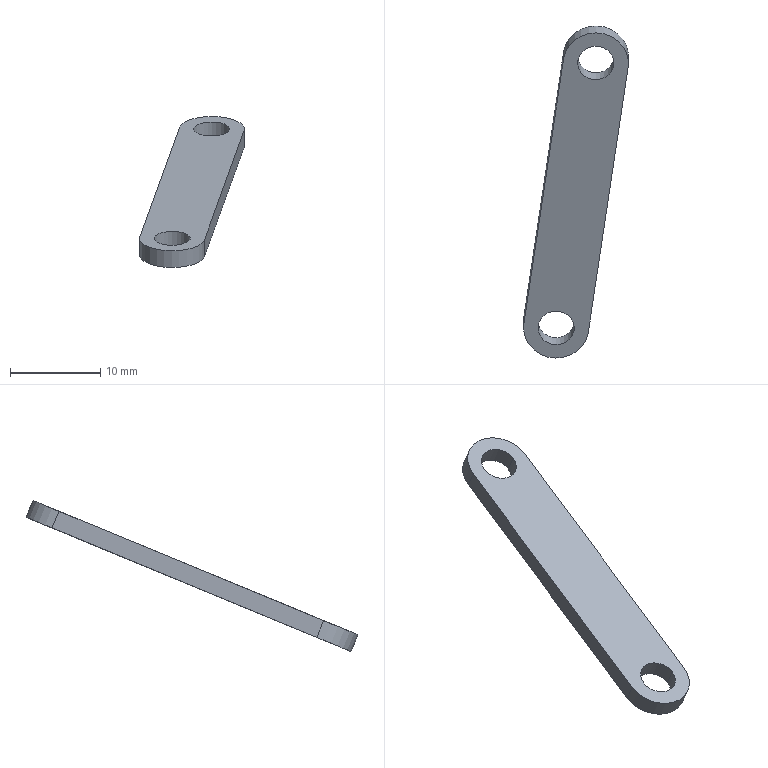Component | SolidWorks | Long Arm-1 | 1 solid | 10 faces | box 11.59 x 36.71 x 16.7 mm | volume 492 mm3 | cylinder 6 | plane 4 | commonest cylinder face diameters 4 x4 7.2 x2
build123d program:
from build123d import *

# Parameters (mm, degrees)
SKETCH2_R           = 5
BOSS_EXTRUDE1_DEPTH = 2.5
SCALE1_SCALE        = 0.4


with BuildPart() as part:
    # Sketch2 → Boss-Extrude1 (new, symmetric)
    with BuildSketch(Plane(origin=(0, 0, 0), x_dir=(1, 0, 0), z_dir=(0, 1, 0))):
        with BuildLine():
            Line((0, 9), (80, 9))
            ThreePointArc((80, 9), (89, 0), (80, -9))
            Line((80, -9), (0, -9))
            ThreePointArc((0, -9), (-9, 0), (0, 9))
        make_face()
        with Locations(Location((0, 0, 0), (0, 0, 270))):
            Circle(SKETCH2_R, mode=Mode.SUBTRACT)
        with Locations(Location((80, 0, 0), (0, 0, 270))):
            Circle(SKETCH2_R, mode=Mode.SUBTRACT)
    extrude(amount=BOSS_EXTRUDE1_DEPTH, both=True)


with BuildPart() as part_1:
    # Scale1: scaled about (0, 0, 0)
    add(part.part.scale(SCALE1_SCALE))


solid = part_1.part

# Placed as in the assembly
solid = solid.moved(Location((343.013, 24.265, 76.802), (-67.552, -82.111, 180)))
STEP:
#1=CARTESIAN_POINT('',(13.582,0.9604,2.983));
#2=VERTEX_POINT('',#1);
#3=CARTESIAN_POINT('',(13.426,0.9803,2.991));
#4=VERTEX_POINT('',#3);
#5=CARTESIAN_POINT('',(13.504,0.9703,2.987));
#6=DIRECTION('',(0.,0.3818,-0.9242));
#7=DIRECTION('',(-0.9905,0.1268,0.05241));
#8=AXIS2_PLACEMENT_3D('',#5,#6,#7);
#9=CIRCLE('',#8,0.07874);
#10=EDGE_CURVE('',#2,#4,#9,.T.);
#11=ORIENTED_EDGE('',*,*,#10,.T.);
#12=CARTESIAN_POINT('',(13.426,0.9503,3.064));
#13=VERTEX_POINT('',#12);
#14=CARTESIAN_POINT('',(13.426,0.9803,2.991));
#15=DIRECTION('',(-0.,-0.3818,0.9242));
#16=VECTOR('',#15,39.37);
#17=LINE('',#14,#16);
#18=EDGE_CURVE('',#4,#13,#17,.T.);
#19=ORIENTED_EDGE('',*,*,#18,.T.);
#20=CARTESIAN_POINT('',(13.582,0.9303,3.056));
#21=VERTEX_POINT('',#20);
#22=CARTESIAN_POINT('',(13.504,0.9403,3.06));
#23=DIRECTION('',(0.,0.3818,-0.9242));
#24=DIRECTION('',(-0.9905,0.1268,0.05241));
#25=AXIS2_PLACEMENT_3D('',#22,#23,#24);
#26=CIRCLE('',#25,0.07874);
#27=EDGE_CURVE('',#21,#13,#26,.T.);
#28=ORIENTED_EDGE('',*,*,#27,.F.);
#29=CARTESIAN_POINT('',(13.582,0.9604,2.983));
#30=DIRECTION('',(-0.,-0.3818,0.9242));
#31=VECTOR('',#30,39.37);
#32=LINE('',#29,#31);
#33=EDGE_CURVE('',#2,#21,#32,.T.);
#34=ORIENTED_EDGE('',*,*,#33,.F.);
#35=EDGE_LOOP('',(#11,#19,#28,#34));
#36=FACE_OUTER_BOUND('',#35,.T.);
#37=CARTESIAN_POINT('',(13.504,0.9703,2.987));
#38=DIRECTION('',(-0.,-0.3818,0.9242));
#39=DIRECTION('',(0.9905,-0.1268,-0.05241));
#40=AXIS2_PLACEMENT_3D('',#37,#38,#39);
#41=CYLINDRICAL_SURFACE('',#40,0.07874);
#42=ADVANCED_FACE('',(#36),#41,.F.);
#43=CARTESIAN_POINT('',(13.41,-0.193,2.507));
#44=VERTEX_POINT('',#43);
#45=CARTESIAN_POINT('',(13.254,-0.173,2.515));
#46=VERTEX_POINT('',#45);
#47=CARTESIAN_POINT('',(13.332,-0.183,2.511));
#48=DIRECTION('',(0.,0.3818,-0.9242));
#49=DIRECTION('',(-0.9905,0.1268,0.05241));
#50=AXIS2_PLACEMENT_3D('',#47,#48,#49);
#51=CIRCLE('',#50,0.07874);
#52=EDGE_CURVE('',#44,#46,#51,.T.);
#53=ORIENTED_EDGE('',*,*,#52,.T.);
#54=CARTESIAN_POINT('',(13.254,-0.2031,2.588));
#55=VERTEX_POINT('',#54);
#56=CARTESIAN_POINT('',(13.254,-0.173,2.515));
#57=DIRECTION('',(-0.,-0.3818,0.9242));
#58=VECTOR('',#57,39.37);
#59=LINE('',#56,#58);
#60=EDGE_CURVE('',#46,#55,#59,.T.);
#61=ORIENTED_EDGE('',*,*,#60,.T.);
#62=CARTESIAN_POINT('',(13.41,-0.2231,2.579));
#63=VERTEX_POINT('',#62);
#64=CARTESIAN_POINT('',(13.332,-0.2131,2.584));
#65=DIRECTION('',(0.,0.3818,-0.9242));
#66=DIRECTION('',(-0.9905,0.1268,0.05241));
#67=AXIS2_PLACEMENT_3D('',#64,#65,#66);
#68=CIRCLE('',#67,0.07874);
#69=EDGE_CURVE('',#63,#55,#68,.T.);
#70=ORIENTED_EDGE('',*,*,#69,.F.);
#71=CARTESIAN_POINT('',(13.41,-0.193,2.507));
#72=DIRECTION('',(-0.,-0.3818,0.9242));
#73=VECTOR('',#72,39.37);
#74=LINE('',#71,#73);
#75=EDGE_CURVE('',#44,#63,#74,.T.);
#76=ORIENTED_EDGE('',*,*,#75,.F.);
#77=EDGE_LOOP('',(#53,#61,#70,#76));
#78=FACE_OUTER_BOUND('',#77,.T.);
#79=CARTESIAN_POINT('',(13.332,-0.183,2.511));
#80=DIRECTION('',(-0.,-0.3818,0.9242));
#81=DIRECTION('',(0.9905,-0.1268,-0.05241));
#82=AXIS2_PLACEMENT_3D('',#79,#80,#81);
#83=CYLINDRICAL_SURFACE('',#82,0.07874);
#84=ADVANCED_FACE('',(#78),#83,.F.);
#85=ORIENTED_EDGE('',*,*,#52,.F.);
#86=CARTESIAN_POINT('',(13.332,-0.183,2.511));
#87=DIRECTION('',(0.,0.3818,-0.9242));
#88=DIRECTION('',(-0.9905,0.1268,0.05241));
#89=AXIS2_PLACEMENT_3D('',#86,#87,#88);
#90=CIRCLE('',#89,0.07874);
#91=EDGE_CURVE('',#46,#44,#90,.T.);
#92=ORIENTED_EDGE('',*,*,#91,.F.);
#93=EDGE_LOOP('',(#85,#92));
#94=FACE_BOUND('',#93,.T.);
#95=CARTESIAN_POINT('',(13.472,-0.201,2.503));
#96=VERTEX_POINT('',#95);
#97=CARTESIAN_POINT('',(13.191,-0.165,2.518));
#98=VERTEX_POINT('',#97);
#99=CARTESIAN_POINT('',(13.332,-0.183,2.511));
#100=DIRECTION('',(0.,0.3818,-0.9242));
#101=DIRECTION('',(-0.9905,0.1268,0.05241));
#102=AXIS2_PLACEMENT_3D('',#99,#100,#101);
#103=CIRCLE('',#102,0.1417);
#104=EDGE_CURVE('',#96,#98,#103,.T.);
#105=ORIENTED_EDGE('',*,*,#104,.T.);
#106=CARTESIAN_POINT('',(13.364,0.9883,2.995));
#107=VERTEX_POINT('',#106);
#108=CARTESIAN_POINT('',(13.191,-0.165,2.518));
#109=DIRECTION('',(0.1372,0.9155,0.3782));
#110=VECTOR('',#109,39.37);
#111=LINE('',#108,#110);
#112=EDGE_CURVE('',#98,#107,#111,.T.);
#113=ORIENTED_EDGE('',*,*,#112,.T.);
#114=CARTESIAN_POINT('',(13.645,0.9524,2.98));
#115=VERTEX_POINT('',#114);
#116=CARTESIAN_POINT('',(13.504,0.9703,2.987));
#117=DIRECTION('',(0.,0.3818,-0.9242));
#118=DIRECTION('',(-0.9905,0.1268,0.05241));
#119=AXIS2_PLACEMENT_3D('',#116,#117,#118);
#120=CIRCLE('',#119,0.1417);
#121=EDGE_CURVE('',#107,#115,#120,.T.);
#122=ORIENTED_EDGE('',*,*,#121,.T.);
#123=CARTESIAN_POINT('',(13.472,-0.201,2.503));
#124=DIRECTION('',(-0.1372,-0.9155,-0.3782));
#125=VECTOR('',#124,39.37);
#126=LINE('',#123,#125);
#127=EDGE_CURVE('',#115,#96,#126,.T.);
#128=ORIENTED_EDGE('',*,*,#127,.T.);
#129=EDGE_LOOP('',(#105,#113,#122,#128));
#130=FACE_OUTER_BOUND('',#129,.T.);
#131=ORIENTED_EDGE('',*,*,#10,.F.);
#132=CARTESIAN_POINT('',(13.504,0.9703,2.987));
#133=DIRECTION('',(0.,0.3818,-0.9242));
#134=DIRECTION('',(-0.9905,0.1268,0.05241));
#135=AXIS2_PLACEMENT_3D('',#132,#133,#134);
#136=CIRCLE('',#135,0.07874);
#137=EDGE_CURVE('',#4,#2,#136,.T.);
#138=ORIENTED_EDGE('',*,*,#137,.F.);
#139=EDGE_LOOP('',(#131,#138));
#140=FACE_BOUND('',#139,.T.);
#141=CARTESIAN_POINT('',(13.332,-0.183,2.511));
#142=DIRECTION('',(0.,0.3818,-0.9242));
#143=DIRECTION('',(-0.9905,0.1268,0.05241));
#144=AXIS2_PLACEMENT_3D('',#141,#142,#143);
#145=PLANE('',#144);
#146=ADVANCED_FACE('',(#94,#130,#140),#145,.T.);
#147=CARTESIAN_POINT('',(13.472,-0.2311,2.576));
#148=VERTEX_POINT('',#147);
#149=CARTESIAN_POINT('',(13.191,-0.1951,2.591));
#150=VERTEX_POINT('',#149);
#151=CARTESIAN_POINT('',(13.332,-0.2131,2.584));
#152=DIRECTION('',(0.,0.3818,-0.9242));
#153=DIRECTION('',(-0.9905,0.1268,0.05241));
#154=AXIS2_PLACEMENT_3D('',#151,#152,#153);
#155=CIRCLE('',#154,0.1417);
#156=EDGE_CURVE('',#148,#150,#155,.T.);
#157=ORIENTED_EDGE('',*,*,#156,.F.);
#158=CARTESIAN_POINT('',(13.645,0.9223,3.053));
#159=VERTEX_POINT('',#158);
#160=CARTESIAN_POINT('',(13.472,-0.2311,2.576));
#161=DIRECTION('',(-0.1372,-0.9155,-0.3782));
#162=VECTOR('',#161,39.37);
#163=LINE('',#160,#162);
#164=EDGE_CURVE('',#159,#148,#163,.T.);
#165=ORIENTED_EDGE('',*,*,#164,.F.);
#166=CARTESIAN_POINT('',(13.364,0.9583,3.068));
#167=VERTEX_POINT('',#166);
#168=CARTESIAN_POINT('',(13.504,0.9403,3.06));
#169=DIRECTION('',(0.,0.3818,-0.9242));
#170=DIRECTION('',(-0.9905,0.1268,0.05241));
#171=AXIS2_PLACEMENT_3D('',#168,#169,#170);
#172=CIRCLE('',#171,0.1417);
#173=EDGE_CURVE('',#167,#159,#172,.T.);
#174=ORIENTED_EDGE('',*,*,#173,.F.);
#175=CARTESIAN_POINT('',(13.191,-0.1951,2.591));
#176=DIRECTION('',(0.1372,0.9155,0.3782));
#177=VECTOR('',#176,39.37);
#178=LINE('',#175,#177);
#179=EDGE_CURVE('',#150,#167,#178,.T.);
#180=ORIENTED_EDGE('',*,*,#179,.F.);
#181=EDGE_LOOP('',(#157,#165,#174,#180));
#182=FACE_OUTER_BOUND('',#181,.T.);
#183=ORIENTED_EDGE('',*,*,#69,.T.);
#184=CARTESIAN_POINT('',(13.332,-0.2131,2.584));
#185=DIRECTION('',(0.,0.3818,-0.9242));
#186=DIRECTION('',(-0.9905,0.1268,0.05241));
#187=AXIS2_PLACEMENT_3D('',#184,#185,#186);
#188=CIRCLE('',#187,0.07874);
#189=EDGE_CURVE('',#55,#63,#188,.T.);
#190=ORIENTED_EDGE('',*,*,#189,.T.);
#191=EDGE_LOOP('',(#183,#190));
#192=FACE_BOUND('',#191,.T.);
#193=ORIENTED_EDGE('',*,*,#27,.T.);
#194=CARTESIAN_POINT('',(13.504,0.9403,3.06));
#195=DIRECTION('',(0.,0.3818,-0.9242));
#196=DIRECTION('',(-0.9905,0.1268,0.05241));
#197=AXIS2_PLACEMENT_3D('',#194,#195,#196);
#198=CIRCLE('',#197,0.07874);
#199=EDGE_CURVE('',#13,#21,#198,.T.);
#200=ORIENTED_EDGE('',*,*,#199,.T.);
#201=EDGE_LOOP('',(#193,#200));
#202=FACE_BOUND('',#201,.T.);
#203=CARTESIAN_POINT('',(13.332,-0.2131,2.584));
#204=DIRECTION('',(0.,0.3818,-0.9242));
#205=DIRECTION('',(-0.9905,0.1268,0.05241));
#206=AXIS2_PLACEMENT_3D('',#203,#204,#205);
#207=PLANE('',#206);
#208=ADVANCED_FACE('',(#182,#192,#202),#207,.F.);
#209=ORIENTED_EDGE('',*,*,#156,.T.);
#210=CARTESIAN_POINT('',(13.191,-0.165,2.518));
#211=DIRECTION('',(-0.,-0.3818,0.9242));
#212=VECTOR('',#211,39.37);
#213=LINE('',#210,#212);
#214=EDGE_CURVE('',#98,#150,#213,.T.);
#215=ORIENTED_EDGE('',*,*,#214,.F.);
#216=ORIENTED_EDGE('',*,*,#104,.F.);
#217=CARTESIAN_POINT('',(13.472,-0.201,2.503));
#218=DIRECTION('',(-0.,-0.3818,0.9242));
#219=VECTOR('',#218,39.37);
#220=LINE('',#217,#219);
#221=EDGE_CURVE('',#96,#148,#220,.T.);
#222=ORIENTED_EDGE('',*,*,#221,.T.);
#223=EDGE_LOOP('',(#209,#215,#216,#222));
#224=FACE_OUTER_BOUND('',#223,.T.);
#225=CARTESIAN_POINT('',(13.332,-0.183,2.511));
#226=DIRECTION('',(-0.,-0.3818,0.9242));
#227=DIRECTION('',(0.9905,-0.1268,-0.05241));
#228=AXIS2_PLACEMENT_3D('',#225,#226,#227);
#229=CYLINDRICAL_SURFACE('',#228,0.1417);
#230=ADVANCED_FACE('',(#224),#229,.T.);
#231=ORIENTED_EDGE('',*,*,#179,.T.);
#232=CARTESIAN_POINT('',(13.364,0.9883,2.995));
#233=DIRECTION('',(-0.,-0.3818,0.9242));
#234=VECTOR('',#233,39.37);
#235=LINE('',#232,#234);
#236=EDGE_CURVE('',#107,#167,#235,.T.);
#237=ORIENTED_EDGE('',*,*,#236,.F.);
#238=ORIENTED_EDGE('',*,*,#112,.F.);
#239=ORIENTED_EDGE('',*,*,#214,.T.);
#240=EDGE_LOOP('',(#231,#237,#238,#239));
#241=FACE_OUTER_BOUND('',#240,.T.);
#242=CARTESIAN_POINT('',(13.191,-0.165,2.518));
#243=DIRECTION('',(0.9905,-0.1268,-0.05241));
#244=DIRECTION('',(-0.1372,-0.9155,-0.3782));
#245=AXIS2_PLACEMENT_3D('',#242,#243,#244);
#246=PLANE('',#245);
#247=ADVANCED_FACE('',(#241),#246,.F.);
#248=ORIENTED_EDGE('',*,*,#173,.T.);
#249=CARTESIAN_POINT('',(13.645,0.9524,2.98));
#250=DIRECTION('',(-0.,-0.3818,0.9242));
#251=VECTOR('',#250,39.37);
#252=LINE('',#249,#251);
#253=EDGE_CURVE('',#115,#159,#252,.T.);
#254=ORIENTED_EDGE('',*,*,#253,.F.);
#255=ORIENTED_EDGE('',*,*,#121,.F.);
#256=ORIENTED_EDGE('',*,*,#236,.T.);
#257=EDGE_LOOP('',(#248,#254,#255,#256));
#258=FACE_OUTER_BOUND('',#257,.T.);
#259=CARTESIAN_POINT('',(13.504,0.9703,2.987));
#260=DIRECTION('',(-0.,-0.3818,0.9242));
#261=DIRECTION('',(0.9905,-0.1268,-0.05241));
#262=AXIS2_PLACEMENT_3D('',#259,#260,#261);
#263=CYLINDRICAL_SURFACE('',#262,0.1417);
#264=ADVANCED_FACE('',(#258),#263,.T.);
#265=ORIENTED_EDGE('',*,*,#164,.T.);
#266=ORIENTED_EDGE('',*,*,#221,.F.);
#267=ORIENTED_EDGE('',*,*,#127,.F.);
#268=ORIENTED_EDGE('',*,*,#253,.T.);
#269=EDGE_LOOP('',(#265,#266,#267,#268));
#270=FACE_OUTER_BOUND('',#269,.T.);
#271=CARTESIAN_POINT('',(13.472,-0.201,2.503));
#272=DIRECTION('',(-0.9905,0.1268,0.05241));
#273=DIRECTION('',(0.1372,0.9155,0.3782));
#274=AXIS2_PLACEMENT_3D('',#271,#272,#273);
#275=PLANE('',#274);
#276=ADVANCED_FACE('',(#270),#275,.F.);
#277=ORIENTED_EDGE('',*,*,#60,.F.);
#278=ORIENTED_EDGE('',*,*,#91,.T.);
#279=ORIENTED_EDGE('',*,*,#75,.T.);
#280=ORIENTED_EDGE('',*,*,#189,.F.);
#281=EDGE_LOOP('',(#277,#278,#279,#280));
#282=FACE_OUTER_BOUND('',#281,.T.);
#283=CARTESIAN_POINT('',(13.332,-0.183,2.511));
#284=DIRECTION('',(-0.,-0.3818,0.9242));
#285=DIRECTION('',(0.9905,-0.1268,-0.05241));
#286=AXIS2_PLACEMENT_3D('',#283,#284,#285);
#287=CYLINDRICAL_SURFACE('',#286,0.07874);
#288=ADVANCED_FACE('',(#282),#287,.F.);
#289=ORIENTED_EDGE('',*,*,#18,.F.);
#290=ORIENTED_EDGE('',*,*,#137,.T.);
#291=ORIENTED_EDGE('',*,*,#33,.T.);
#292=ORIENTED_EDGE('',*,*,#199,.F.);
#293=EDGE_LOOP('',(#289,#290,#291,#292));
#294=FACE_OUTER_BOUND('',#293,.T.);
#295=CARTESIAN_POINT('',(13.504,0.9703,2.987));
#296=DIRECTION('',(-0.,-0.3818,0.9242));
#297=DIRECTION('',(0.9905,-0.1268,-0.05241));
#298=AXIS2_PLACEMENT_3D('',#295,#296,#297);
#299=CYLINDRICAL_SURFACE('',#298,0.07874);
#300=ADVANCED_FACE('',(#294),#299,.F.);
#301=CLOSED_SHELL('',(#42,#84,#146,#208,#230,#247,#264,#276,#288,#300));
#302=MANIFOLD_SOLID_BREP('',#301);
#303=CARTESIAN_POINT('',(0.,0.,0.));
#304=DIRECTION('',(0.,0.,1.));
#305=DIRECTION('',(1.,0.,0.));
#306=AXIS2_PLACEMENT_3D('',#303,#304,#305);
#307=(LENGTH_UNIT()NAMED_UNIT(*)SI_UNIT($,.METRE.));
#308=LENGTH_MEASURE_WITH_UNIT(LENGTH_MEASURE(0.0254),#307);
#309=DIMENSIONAL_EXPONENTS(1.,0.,0.,0.,0.,0.,0.);
#310=(CONVERSION_BASED_UNIT('',#308)LENGTH_UNIT()NAMED_UNIT(#309));
#311=UNCERTAINTY_MEASURE_WITH_UNIT(LENGTH_MEASURE(0.00001),#310,'','');
#312=(NAMED_UNIT(*)PLANE_ANGLE_UNIT()SI_UNIT($,.RADIAN.));
#313=(NAMED_UNIT(*)SI_UNIT($,.STERADIAN.)SOLID_ANGLE_UNIT());
#314=(GEOMETRIC_REPRESENTATION_CONTEXT(3)GLOBAL_UNCERTAINTY_ASSIGNED_CONTEXT((#311))GLOBAL_UNIT_ASSIGNED_CONTEXT((#310,#312,#313))REPRESENTATION_CONTEXT('',''));
#315=ADVANCED_BREP_SHAPE_REPRESENTATION('',(#302,#306),#314);
#316=COLOUR_RGB('',0.7922,0.8196,0.9333);
#317=FILL_AREA_STYLE_COLOUR('',#316);
#318=FILL_AREA_STYLE('',(#317));
#319=SURFACE_STYLE_FILL_AREA(#318);
#320=SURFACE_SIDE_STYLE('',(#319));
#321=SURFACE_STYLE_USAGE(.BOTH.,#320);
#322=PRESENTATION_STYLE_ASSIGNMENT((#321));
#323=STYLED_ITEM('',(#322),#302);
#324=(LENGTH_UNIT()NAMED_UNIT(*)SI_UNIT($,.METRE.));
#325=LENGTH_MEASURE_WITH_UNIT(LENGTH_MEASURE(0.0254),#324);
#326=DIMENSIONAL_EXPONENTS(1.,0.,0.,0.,0.,0.,0.);
#327=(CONVERSION_BASED_UNIT('',#325)LENGTH_UNIT()NAMED_UNIT(#326));
#328=UNCERTAINTY_MEASURE_WITH_UNIT(LENGTH_MEASURE(0.00001),#327,'','');
#329=(NAMED_UNIT(*)PLANE_ANGLE_UNIT()SI_UNIT($,.RADIAN.));
#330=(NAMED_UNIT(*)SI_UNIT($,.STERADIAN.)SOLID_ANGLE_UNIT());
#331=(GEOMETRIC_REPRESENTATION_CONTEXT(3)GLOBAL_UNCERTAINTY_ASSIGNED_CONTEXT((#328))GLOBAL_UNIT_ASSIGNED_CONTEXT((#327,#329,#330))REPRESENTATION_CONTEXT('',''));
#332=MECHANICAL_DESIGN_GEOMETRIC_PRESENTATION_REPRESENTATION('',(#323),#331);
#333=PRESENTATION_LAYER_ASSIGNMENT('','',(#323));